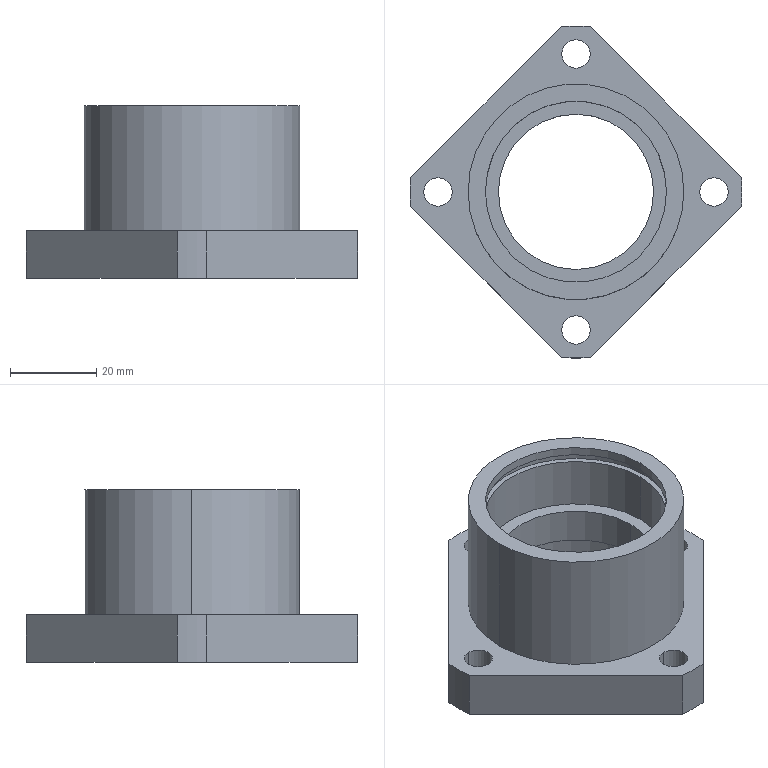Component | SolidWorks | Q1-A12-S21-Q1A.SLDASQ-1_Q1-BGSBB6004ZZ-40.sldasQ-1_Q1-BGSBB6004ZZ-40_h-1 | 1 solid | 54 faces | box 77 x 77 x 40 mm | volume 38671 mm3 | cylinder 37 | plane 17 | commonest cylinder face diameters 11 x8 6.6 x8 42 x8 77 x5 44.5 x4 36 x2 50 x2
build123d program:
from build123d import *

# Parameters (mm, degrees)
LPATTERN1_COUNT      = 2
LPATTERN1_PITCH      = 45.255
LPATTERN1_COUNT_DIR2 = 2
LPATTERN1_PITCH_DIR2 = 45.255
SKETCH5_R            = 59
CUT_EXTRUDE1_DEPTH   = 11


with BuildPart() as part:
    # Sketch1 → Revolve1 (revolve)
    with BuildSketch(Plane.XY, mode=Mode.PRIVATE) as revolve1_sk:
        Polygon((-40, 0), (-40, 25), (-11, 25), (-11, 38.5), (0, 38.5), (0, 0), align=None)
    revolve(revolve1_sk.sketch.rotate(Axis((0, 0, 0), (-1, 0, 0)), 270), axis=Axis((0, 0, 0), (-1, 0, 0)))

    # Sketch2 → Cut-Revolve1 (revolve, cut)
    with BuildSketch(Plane.XY, mode=Mode.PRIVATE) as cut_revolve1_sk:
        Polygon((-40, 0), (-40, 21), (-38, 21), (-38, 22.25), (-36.05, 22.25), (-36.05, 21), (-24.05, 21), (-24.05, 18), (-15.95, 18), (-15.95, 21), (-3.95, 21), (-3.95, 22.25), (-2, 22.25), (-2, 21), (0, 21), (0, 0), align=None)
    revolve(cut_revolve1_sk.sketch.rotate(Axis((0, 0, 0), (-1, 0, 0)), 270), axis=Axis((0, 0, 0), (-1, 0, 0)), mode=Mode.SUBTRACT)

    # Sketch3 → Cut-Revolve2 (revolve, cut)
    with BuildSketch(Plane.XY, mode=Mode.PRIVATE) as cut_revolve2_sk:
        Polygon((-11, 32), (-11, 35.3), (-6.1, 35.3), (-6.1, 37.5), (0, 37.5), (0, 32), align=None)
    cut_revolve2 = revolve(cut_revolve2_sk.sketch.rotate(Axis((0, 32, 0), (-1, 0, 0)), 180), axis=Axis((0, 32, 0), (-1, 0, 0)), mode=Mode.SUBTRACT)

    # LPattern1: Cut-Revolve2 2 × 2
    with Locations(*[Vector(0, -0.7071, 0.7071) * (i * LPATTERN1_PITCH) + Vector(0, -0.7071, -0.7071) * (j * LPATTERN1_PITCH_DIR2) for i in range(LPATTERN1_COUNT) for j in range(LPATTERN1_COUNT_DIR2) if (i, j) != (0, 0)]):
        add(cut_revolve2, mode=Mode.SUBTRACT)

    # Sketch5 → Cut-Extrude1 (cut)
    with BuildSketch(Plane(origin=(0, 0, 0), x_dir=(0, 0, -1), z_dir=(1, 0, 0))):
        Circle(SKETCH5_R)
        Polygon((-41.719, 0), (0, -41.719), (41.719, 0), (0, 41.719), align=None, mode=Mode.SUBTRACT)
    extrude(amount=-CUT_EXTRUDE1_DEPTH, mode=Mode.SUBTRACT)


solid = part.part

# Placed as in the assembly
solid = solid.moved(Location((0, 0, -173.5), (0, 90, 0)))